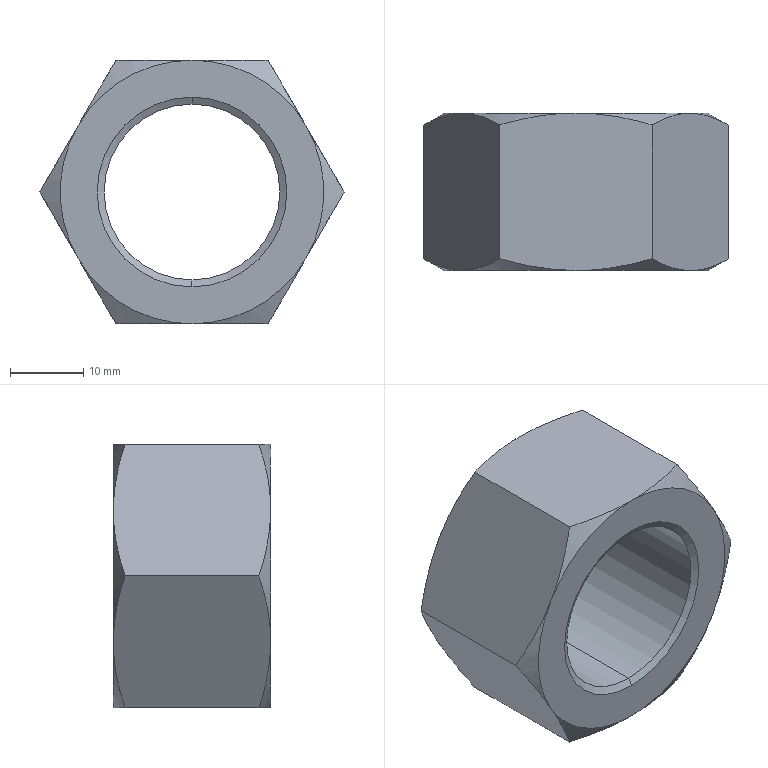Component | SolidWorks | GB_T6170-2015[Type1HexNutM24]-3 | 1 solid | 26 faces | box 41.57 x 21.5 x 36 mm | volume 14263 mm3 | cone 16 | plane 8 | cylinder 2 | commonest cylinder face diameters 24 x2
build123d program:
from build123d import *

# Parameters (mm, degrees)
SKETCH3_R               = 10.376
BOSS_EXTRUDE1_DEPTH     = 21.5
SKETCH5_R               = 29.663
SKETCH5_R_2             = 18
CUT_EXTRUDE1_2_DEPTH    = 4.3
CUT_EXTRUDE1_2_DRAFT    = -60
SKETCH7_R               = 29.663
SKETCH7_R_2             = 18
CUT_EXTRUDE2_DEPTH      = 4.3
CUT_EXTRUDE2_DRAFT      = -60
CUT_EXTRUDE1_DEPTH      = 35.903
CUT_EXTRUDE1_DEPTH_BACK = 35.903
SKETCH1_R               = 12


with BuildPart() as part:
    # Sketch3 → Boss-Extrude1 (new body)
    with BuildSketch(Plane.XY):
        Polygon((0, 20.785), (-18, 10.392), (-18, -10.392), (0, -20.785), (18, -10.392), (18, 10.392), align=None)
        Circle(SKETCH3_R, mode=Mode.SUBTRACT)
    extrude(amount=-BOSS_EXTRUDE1_DEPTH)

    # Sketch4 → Cut-Revolve1 (revolve, cut)
    with BuildSketch(Plane(origin=(0, 0, 0), x_dir=(0, 0, -1), z_dir=(1, 0, 0)), mode=Mode.PRIVATE) as cut_revolve1_sk:
        Polygon((0, 12.95), (1.486, 10.376), (1.486, 0), (0, 0), align=None)
        Polygon((21.5, 0), (21.5, 12.95), (20.014, 10.376), (20.014, 0), align=None)
    revolve(cut_revolve1_sk.sketch.rotate(Axis((0, 0, 0), (0, 0, -1)), 90), axis=Axis((0, 0, 0), (0, 0, -1)), mode=Mode.SUBTRACT)


with BuildPart() as cut_extrude1_2_tool:
    # Sketch5 → Cut-Extrude1_2 (with draft: the straight prism first)
    with BuildSketch(Plane.XY):
        Circle(SKETCH5_R)
        Circle(SKETCH5_R_2, mode=Mode.SUBTRACT)
    extrude(amount=-CUT_EXTRUDE1_2_DEPTH)
    # Cut-Extrude1_2: the draft: its side faces are tilted about the plane it starts from
    cut_extrude1_2_sides = [cut_extrude1_2_tool.faces().sort_by_distance(p)[0] for p in [
        (-29.663, 0, -2.15),
        (-18, 0, -2.15),
    ]]
    draft(cut_extrude1_2_sides, Plane.XY, CUT_EXTRUDE1_2_DRAFT)


with BuildPart() as part_1:
    add(part.part)

    # Cut-Extrude1_2: cut by cut_extrude1_2_tool
    add(cut_extrude1_2_tool.part, mode=Mode.SUBTRACT)


with BuildPart() as cut_extrude2_tool:
    # Sketch7 → Cut-Extrude2 (with draft: the straight prism first)
    with BuildSketch(Plane(origin=(0, 0, -21.5), x_dir=(-1, 0, 0), z_dir=(0, 0, -1))):
        Circle(SKETCH7_R)
        Circle(SKETCH7_R_2, mode=Mode.SUBTRACT)
    extrude(amount=-CUT_EXTRUDE2_DEPTH)
    # Cut-Extrude2: the draft: its side faces are tilted about the plane it starts from
    cut_extrude2_sides = [cut_extrude2_tool.faces().sort_by_distance(p)[0] for p in [
        (29.663, 0, -19.35),
        (18, 0, -19.35),
    ]]
    draft(cut_extrude2_sides, Plane(origin=(0, 0, -21.5), x_dir=(-1, 0, 0), z_dir=(0, 0, -1)), CUT_EXTRUDE2_DRAFT)


with BuildPart() as part_2:
    add(part_1.part)

    # Cut-Extrude2: cut by cut_extrude2_tool
    add(cut_extrude2_tool.part, mode=Mode.SUBTRACT)

    # Sketch1 → Cut-Extrude1 (cut, two sides: drawn at the far end of the back side and taken through both)
    with BuildSketch(Plane.XY.offset(-CUT_EXTRUDE1_DEPTH_BACK)):
        Circle(SKETCH1_R)
    extrude(amount=CUT_EXTRUDE1_DEPTH + CUT_EXTRUDE1_DEPTH_BACK, mode=Mode.SUBTRACT)


solid = part_2.part

# Placed as in the assembly
solid = solid.moved(Location((82.5, 20, 142.894), (90, 0, 90)))
STEP:
#1=COLOUR_RGB('',0.7922,0.8196,0.9333);
#2=FILL_AREA_STYLE_COLOUR('',#1);
#3=FILL_AREA_STYLE('',(#2));
#4=SURFACE_STYLE_FILL_AREA(#3);
#5=SURFACE_SIDE_STYLE('',(#4));
#6=SURFACE_STYLE_USAGE(.BOTH.,#5);
#7=PRESENTATION_STYLE_ASSIGNMENT((#6));
#8=CARTESIAN_POINT('',(3.248,0.809,5.153));
#9=VERTEX_POINT('',#8);
#10=CARTESIAN_POINT('',(3.248,0.809,6.098));
#11=VERTEX_POINT('',#10);
#12=CARTESIAN_POINT('',(3.248,0.809,5.626));
#13=DIRECTION('',(0.,-1.,0.));
#14=DIRECTION('',(0.,0.,1.));
#15=AXIS2_PLACEMENT_3D('',#12,#13,#14);
#16=CIRCLE('',#15,0.4724);
#17=EDGE_CURVE('',#9,#11,#16,.T.);
#18=ORIENTED_EDGE('',*,*,#17,.T.);
#19=CARTESIAN_POINT('',(3.248,1.612,6.098));
#20=VERTEX_POINT('',#19);
#21=CARTESIAN_POINT('',(3.248,0.7874,6.098));
#22=DIRECTION('',(0.,1.,0.));
#23=VECTOR('',#22,39.37);
#24=LINE('',#21,#23);
#25=EDGE_CURVE('',#11,#20,#24,.T.);
#26=ORIENTED_EDGE('',*,*,#25,.T.);
#27=CARTESIAN_POINT('',(3.248,1.612,5.153));
#28=VERTEX_POINT('',#27);
#29=CARTESIAN_POINT('',(3.248,1.612,5.626));
#30=DIRECTION('',(0.,1.,0.));
#31=DIRECTION('',(-0.,0.,-1.));
#32=AXIS2_PLACEMENT_3D('',#29,#30,#31);
#33=CIRCLE('',#32,0.4724);
#34=EDGE_CURVE('',#20,#28,#33,.T.);
#35=ORIENTED_EDGE('',*,*,#34,.T.);
#36=CARTESIAN_POINT('',(3.248,0.7874,5.153));
#37=DIRECTION('',(0.,1.,0.));
#38=VECTOR('',#37,39.37);
#39=LINE('',#36,#38);
#40=EDGE_CURVE('',#9,#28,#39,.T.);
#41=ORIENTED_EDGE('',*,*,#40,.F.);
#42=EDGE_LOOP('',(#18,#26,#35,#41));
#43=FACE_OUTER_BOUND('',#42,.T.);
#44=CARTESIAN_POINT('',(3.248,0.7874,5.626));
#45=DIRECTION('',(0.,1.,0.));
#46=DIRECTION('',(-0.,0.,-1.));
#47=AXIS2_PLACEMENT_3D('',#44,#45,#46);
#48=CYLINDRICAL_SURFACE('',#47,0.4724);
#49=ADVANCED_FACE('',(#43),#48,.F.);
#50=ORIENTED_EDGE('',*,*,#17,.F.);
#51=CARTESIAN_POINT('',(3.248,0.7874,5.116));
#52=VERTEX_POINT('',#51);
#53=CARTESIAN_POINT('',(3.248,0.7874,5.116));
#54=DIRECTION('',(-0.,-0.5,-0.866));
#55=VECTOR('',#54,39.37);
#56=LINE('',#53,#55);
#57=EDGE_CURVE('',#9,#52,#56,.T.);
#58=ORIENTED_EDGE('',*,*,#57,.T.);
#59=CARTESIAN_POINT('',(3.248,0.7874,6.136));
#60=VERTEX_POINT('',#59);
#61=CARTESIAN_POINT('',(3.248,0.7874,5.626));
#62=DIRECTION('',(0.,1.,0.));
#63=DIRECTION('',(-0.,0.,-1.));
#64=AXIS2_PLACEMENT_3D('',#61,#62,#63);
#65=CIRCLE('',#64,0.5098);
#66=EDGE_CURVE('',#60,#52,#65,.T.);
#67=ORIENTED_EDGE('',*,*,#66,.F.);
#68=CARTESIAN_POINT('',(3.248,0.7874,6.136));
#69=DIRECTION('',(0.,-0.5,0.866));
#70=VECTOR('',#69,39.37);
#71=LINE('',#68,#70);
#72=EDGE_CURVE('',#11,#60,#71,.T.);
#73=ORIENTED_EDGE('',*,*,#72,.F.);
#74=EDGE_LOOP('',(#50,#58,#67,#73));
#75=FACE_OUTER_BOUND('',#74,.T.);
#76=CARTESIAN_POINT('',(3.248,0.7874,5.626));
#77=DIRECTION('',(0.,-1.,0.));
#78=DIRECTION('',(0.,0.,1.));
#79=AXIS2_PLACEMENT_3D('',#76,#77,#78);
#80=CONICAL_SURFACE('',#79,0.5098,1.047);
#81=ADVANCED_FACE('',(#75),#80,.F.);
#82=ORIENTED_EDGE('',*,*,#34,.F.);
#83=CARTESIAN_POINT('',(3.248,1.634,6.136));
#84=VERTEX_POINT('',#83);
#85=CARTESIAN_POINT('',(3.248,1.575,6.034));
#86=DIRECTION('',(0.,0.5,0.866));
#87=VECTOR('',#86,39.37);
#88=LINE('',#85,#87);
#89=EDGE_CURVE('',#20,#84,#88,.T.);
#90=ORIENTED_EDGE('',*,*,#89,.T.);
#91=CARTESIAN_POINT('',(3.248,1.634,5.116));
#92=VERTEX_POINT('',#91);
#93=CARTESIAN_POINT('',(3.248,1.634,5.626));
#94=DIRECTION('',(0.,1.,0.));
#95=DIRECTION('',(-0.,0.,-1.));
#96=AXIS2_PLACEMENT_3D('',#93,#94,#95);
#97=CIRCLE('',#96,0.5098);
#98=EDGE_CURVE('',#84,#92,#97,.T.);
#99=ORIENTED_EDGE('',*,*,#98,.T.);
#100=CARTESIAN_POINT('',(3.248,1.575,5.217));
#101=DIRECTION('',(-0.,0.5,-0.866));
#102=VECTOR('',#101,39.37);
#103=LINE('',#100,#102);
#104=EDGE_CURVE('',#28,#92,#103,.T.);
#105=ORIENTED_EDGE('',*,*,#104,.F.);
#106=EDGE_LOOP('',(#82,#90,#99,#105));
#107=FACE_OUTER_BOUND('',#106,.T.);
#108=CARTESIAN_POINT('',(3.248,1.575,5.626));
#109=DIRECTION('',(0.,1.,0.));
#110=DIRECTION('',(-0.,0.,-1.));
#111=AXIS2_PLACEMENT_3D('',#108,#109,#110);
#112=CONICAL_SURFACE('',#111,0.4085,1.047);
#113=ADVANCED_FACE('',(#107),#112,.F.);
#114=CARTESIAN_POINT('',(2.839,0.8507,4.917));
#115=VERTEX_POINT('',#114);
#116=CARTESIAN_POINT('',(2.839,1.571,4.917));
#117=VERTEX_POINT('',#116);
#118=CARTESIAN_POINT('',(2.839,0.7874,4.917));
#119=DIRECTION('',(0.,1.,0.));
#120=VECTOR('',#119,39.37);
#121=LINE('',#118,#120);
#122=EDGE_CURVE('',#115,#117,#121,.T.);
#123=ORIENTED_EDGE('',*,*,#122,.F.);
#124=CARTESIAN_POINT('',(2.634,0.7874,5.271));
#125=VERTEX_POINT('',#124);
#126=CARTESIAN_POINT('',(2.839,0.8507,4.917));
#127=CARTESIAN_POINT('',(2.805,0.8314,4.975));
#128=CARTESIAN_POINT('',(2.772,0.8155,5.033));
#129=CARTESIAN_POINT('',(2.704,0.7934,5.151));
#130=CARTESIAN_POINT('',(2.669,0.7874,5.211));
#131=CARTESIAN_POINT('',(2.634,0.7874,5.271));
#132=B_SPLINE_CURVE_WITH_KNOTS('',3,(#126,#127,#128,#129,#130,#131),.UNSPECIFIED.,.F.,.F.,(4,2,4),(0.00000024,0.005258,0.01052),.UNSPECIFIED.);
#133=EDGE_CURVE('',#115,#125,#132,.T.);
#134=ORIENTED_EDGE('',*,*,#133,.T.);
#135=CARTESIAN_POINT('',(2.43,0.8507,5.626));
#136=VERTEX_POINT('',#135);
#137=CARTESIAN_POINT('',(2.634,0.7874,5.271));
#138=CARTESIAN_POINT('',(2.626,0.7874,5.286));
#139=CARTESIAN_POINT('',(2.617,0.7878,5.302));
#140=CARTESIAN_POINT('',(2.6,0.7892,5.332));
#141=CARTESIAN_POINT('',(2.591,0.7903,5.347));
#142=CARTESIAN_POINT('',(2.565,0.7947,5.391));
#143=CARTESIAN_POINT('',(2.548,0.799,5.421));
#144=CARTESIAN_POINT('',(2.497,0.8155,5.51));
#145=CARTESIAN_POINT('',(2.463,0.8314,5.568));
#146=CARTESIAN_POINT('',(2.43,0.8507,5.626));
#147=B_SPLINE_CURVE_WITH_KNOTS('',3,(#137,#138,#139,#140,#141,#142,#143,#144,#145,#146),.UNSPECIFIED.,.F.,.F.,(4,2,2,2,4),(0.01052,0.01183,0.01313,0.01575,0.02099),.UNSPECIFIED.);
#148=EDGE_CURVE('',#125,#136,#147,.T.);
#149=ORIENTED_EDGE('',*,*,#148,.T.);
#150=CARTESIAN_POINT('',(2.43,1.571,5.626));
#151=VERTEX_POINT('',#150);
#152=CARTESIAN_POINT('',(2.43,0.7874,5.626));
#153=DIRECTION('',(0.,1.,0.));
#154=VECTOR('',#153,39.37);
#155=LINE('',#152,#154);
#156=EDGE_CURVE('',#136,#151,#155,.T.);
#157=ORIENTED_EDGE('',*,*,#156,.T.);
#158=CARTESIAN_POINT('',(2.634,1.634,5.271));
#159=VERTEX_POINT('',#158);
#160=CARTESIAN_POINT('',(2.43,1.571,5.626));
#161=CARTESIAN_POINT('',(2.463,1.59,5.568));
#162=CARTESIAN_POINT('',(2.497,1.606,5.509));
#163=CARTESIAN_POINT('',(2.565,1.628,5.391));
#164=CARTESIAN_POINT('',(2.599,1.634,5.332));
#165=CARTESIAN_POINT('',(2.634,1.634,5.271));
#166=B_SPLINE_CURVE_WITH_KNOTS('',3,(#160,#161,#162,#163,#164,#165),.UNSPECIFIED.,.F.,.F.,(4,2,4),(0.00000024,0.005258,0.01052),.UNSPECIFIED.);
#167=EDGE_CURVE('',#151,#159,#166,.T.);
#168=ORIENTED_EDGE('',*,*,#167,.T.);
#169=CARTESIAN_POINT('',(2.634,1.634,5.271));
#170=CARTESIAN_POINT('',(2.643,1.634,5.256));
#171=CARTESIAN_POINT('',(2.652,1.633,5.241));
#172=CARTESIAN_POINT('',(2.669,1.632,5.211));
#173=CARTESIAN_POINT('',(2.678,1.631,5.196));
#174=CARTESIAN_POINT('',(2.704,1.627,5.151));
#175=CARTESIAN_POINT('',(2.721,1.622,5.122));
#176=CARTESIAN_POINT('',(2.772,1.606,5.033));
#177=CARTESIAN_POINT('',(2.806,1.59,4.975));
#178=CARTESIAN_POINT('',(2.839,1.571,4.917));
#179=B_SPLINE_CURVE_WITH_KNOTS('',3,(#169,#170,#171,#172,#173,#174,#175,#176,#177,#178),.UNSPECIFIED.,.F.,.F.,(4,2,2,2,4),(0.01052,0.01183,0.01313,0.01575,0.02099),.UNSPECIFIED.);
#180=EDGE_CURVE('',#159,#117,#179,.T.);
#181=ORIENTED_EDGE('',*,*,#180,.T.);
#182=EDGE_LOOP('',(#123,#134,#149,#157,#168,#181));
#183=FACE_OUTER_BOUND('',#182,.T.);
#184=CARTESIAN_POINT('',(2.839,0.7874,4.917));
#185=DIRECTION('',(-0.866,0.,-0.5));
#186=DIRECTION('',(-0.5,0.,0.866));
#187=AXIS2_PLACEMENT_3D('',#184,#185,#186);
#188=PLANE('',#187);
#189=ADVANCED_FACE('',(#183),#188,.T.);
#190=CARTESIAN_POINT('',(3.657,0.8507,4.917));
#191=VERTEX_POINT('',#190);
#192=CARTESIAN_POINT('',(3.657,1.571,4.917));
#193=VERTEX_POINT('',#192);
#194=CARTESIAN_POINT('',(3.657,0.7874,4.917));
#195=DIRECTION('',(0.,1.,0.));
#196=VECTOR('',#195,39.37);
#197=LINE('',#194,#196);
#198=EDGE_CURVE('',#191,#193,#197,.T.);
#199=ORIENTED_EDGE('',*,*,#198,.F.);
#200=CARTESIAN_POINT('',(3.248,0.7874,4.917));
#201=VERTEX_POINT('',#200);
#202=CARTESIAN_POINT('',(3.657,0.8507,4.917));
#203=CARTESIAN_POINT('',(3.591,0.8315,4.917));
#204=CARTESIAN_POINT('',(3.522,0.8154,4.917));
#205=CARTESIAN_POINT('',(3.386,0.7933,4.917));
#206=CARTESIAN_POINT('',(3.317,0.7874,4.917));
#207=CARTESIAN_POINT('',(3.248,0.7874,4.917));
#208=B_SPLINE_CURVE_WITH_KNOTS('',3,(#202,#203,#204,#205,#206,#207),.UNSPECIFIED.,.F.,.F.,(4,2,4),(0.01881,0.02407,0.02933),.UNSPECIFIED.);
#209=EDGE_CURVE('',#191,#201,#208,.T.);
#210=ORIENTED_EDGE('',*,*,#209,.T.);
#211=CARTESIAN_POINT('',(3.248,0.7874,4.917));
#212=CARTESIAN_POINT('',(3.213,0.7874,4.917));
#213=CARTESIAN_POINT('',(3.179,0.7889,4.917));
#214=CARTESIAN_POINT('',(3.109,0.7947,4.917));
#215=CARTESIAN_POINT('',(3.075,0.7991,4.917));
#216=CARTESIAN_POINT('',(2.972,0.8157,4.917));
#217=CARTESIAN_POINT('',(2.905,0.8316,4.917));
#218=CARTESIAN_POINT('',(2.839,0.8507,4.917));
#219=B_SPLINE_CURVE_WITH_KNOTS('',3,(#211,#212,#213,#214,#215,#216,#217,#218),.UNSPECIFIED.,.F.,.F.,(4,2,2,4),(0.02933,0.03196,0.03459,0.03985),.UNSPECIFIED.);
#220=EDGE_CURVE('',#201,#115,#219,.T.);
#221=ORIENTED_EDGE('',*,*,#220,.T.);
#222=ORIENTED_EDGE('',*,*,#122,.T.);
#223=CARTESIAN_POINT('',(3.248,1.634,4.917));
#224=VERTEX_POINT('',#223);
#225=CARTESIAN_POINT('',(2.839,1.571,4.917));
#226=CARTESIAN_POINT('',(2.905,1.59,4.917));
#227=CARTESIAN_POINT('',(2.972,1.606,4.917));
#228=CARTESIAN_POINT('',(3.075,1.622,4.917));
#229=CARTESIAN_POINT('',(3.109,1.627,4.917));
#230=CARTESIAN_POINT('',(3.179,1.632,4.917));
#231=CARTESIAN_POINT('',(3.213,1.634,4.917));
#232=CARTESIAN_POINT('',(3.248,1.634,4.917));
#233=B_SPLINE_CURVE_WITH_KNOTS('',3,(#225,#226,#227,#228,#229,#230,#231,#232),.UNSPECIFIED.,.F.,.F.,(4,2,2,4),(0.04624,0.05151,0.05414,0.05678),.UNSPECIFIED.);
#234=EDGE_CURVE('',#117,#224,#233,.T.);
#235=ORIENTED_EDGE('',*,*,#234,.T.);
#236=CARTESIAN_POINT('',(3.248,1.634,4.917));
#237=CARTESIAN_POINT('',(3.317,1.634,4.917));
#238=CARTESIAN_POINT('',(3.386,1.628,4.917));
#239=CARTESIAN_POINT('',(3.522,1.606,4.917));
#240=CARTESIAN_POINT('',(3.591,1.59,4.917));
#241=CARTESIAN_POINT('',(3.657,1.571,4.917));
#242=B_SPLINE_CURVE_WITH_KNOTS('',3,(#236,#237,#238,#239,#240,#241),.UNSPECIFIED.,.F.,.F.,(4,2,4),(0.05678,0.06204,0.0673),.UNSPECIFIED.);
#243=EDGE_CURVE('',#224,#193,#242,.T.);
#244=ORIENTED_EDGE('',*,*,#243,.T.);
#245=EDGE_LOOP('',(#199,#210,#221,#222,#235,#244));
#246=FACE_OUTER_BOUND('',#245,.T.);
#247=CARTESIAN_POINT('',(3.657,0.7874,4.917));
#248=DIRECTION('',(-0.,0.,-1.));
#249=DIRECTION('',(-1.,0.,0.));
#250=AXIS2_PLACEMENT_3D('',#247,#248,#249);
#251=PLANE('',#250);
#252=ADVANCED_FACE('',(#246),#251,.T.);
#253=CARTESIAN_POINT('',(4.066,0.8507,5.626));
#254=VERTEX_POINT('',#253);
#255=CARTESIAN_POINT('',(4.066,1.571,5.626));
#256=VERTEX_POINT('',#255);
#257=CARTESIAN_POINT('',(4.066,0.7874,5.626));
#258=DIRECTION('',(0.,1.,0.));
#259=VECTOR('',#258,39.37);
#260=LINE('',#257,#259);
#261=EDGE_CURVE('',#254,#256,#260,.T.);
#262=ORIENTED_EDGE('',*,*,#261,.F.);
#263=CARTESIAN_POINT('',(3.862,0.7874,5.271));
#264=VERTEX_POINT('',#263);
#265=CARTESIAN_POINT('',(4.066,0.8507,5.626));
#266=CARTESIAN_POINT('',(4.033,0.8314,5.568));
#267=CARTESIAN_POINT('',(3.999,0.8155,5.509));
#268=CARTESIAN_POINT('',(3.931,0.7934,5.391));
#269=CARTESIAN_POINT('',(3.897,0.7874,5.332));
#270=CARTESIAN_POINT('',(3.862,0.7874,5.271));
#271=B_SPLINE_CURVE_WITH_KNOTS('',3,(#265,#266,#267,#268,#269,#270),.UNSPECIFIED.,.F.,.F.,(4,2,4),(0.00000024,0.005258,0.01052),.UNSPECIFIED.);
#272=EDGE_CURVE('',#254,#264,#271,.T.);
#273=ORIENTED_EDGE('',*,*,#272,.T.);
#274=CARTESIAN_POINT('',(3.862,0.7874,5.271));
#275=CARTESIAN_POINT('',(3.853,0.7874,5.256));
#276=CARTESIAN_POINT('',(3.844,0.7878,5.241));
#277=CARTESIAN_POINT('',(3.827,0.7892,5.211));
#278=CARTESIAN_POINT('',(3.818,0.7903,5.196));
#279=CARTESIAN_POINT('',(3.792,0.7947,5.151));
#280=CARTESIAN_POINT('',(3.775,0.799,5.122));
#281=CARTESIAN_POINT('',(3.724,0.8155,5.033));
#282=CARTESIAN_POINT('',(3.691,0.8314,4.975));
#283=CARTESIAN_POINT('',(3.657,0.8507,4.917));
#284=B_SPLINE_CURVE_WITH_KNOTS('',3,(#274,#275,#276,#277,#278,#279,#280,#281,#282,#283),.UNSPECIFIED.,.F.,.F.,(4,2,2,2,4),(0.01052,0.01183,0.01313,0.01575,0.02099),.UNSPECIFIED.);
#285=EDGE_CURVE('',#264,#191,#284,.T.);
#286=ORIENTED_EDGE('',*,*,#285,.T.);
#287=ORIENTED_EDGE('',*,*,#198,.T.);
#288=CARTESIAN_POINT('',(3.862,1.634,5.271));
#289=VERTEX_POINT('',#288);
#290=CARTESIAN_POINT('',(3.657,1.571,4.917));
#291=CARTESIAN_POINT('',(3.691,1.59,4.975));
#292=CARTESIAN_POINT('',(3.724,1.606,5.033));
#293=CARTESIAN_POINT('',(3.792,1.628,5.151));
#294=CARTESIAN_POINT('',(3.827,1.634,5.211));
#295=CARTESIAN_POINT('',(3.862,1.634,5.271));
#296=B_SPLINE_CURVE_WITH_KNOTS('',3,(#290,#291,#292,#293,#294,#295),.UNSPECIFIED.,.F.,.F.,(4,2,4),(0.00000024,0.005258,0.01052),.UNSPECIFIED.);
#297=EDGE_CURVE('',#193,#289,#296,.T.);
#298=ORIENTED_EDGE('',*,*,#297,.T.);
#299=CARTESIAN_POINT('',(3.862,1.634,5.271));
#300=CARTESIAN_POINT('',(3.87,1.634,5.286));
#301=CARTESIAN_POINT('',(3.879,1.633,5.302));
#302=CARTESIAN_POINT('',(3.897,1.632,5.332));
#303=CARTESIAN_POINT('',(3.905,1.631,5.347));
#304=CARTESIAN_POINT('',(3.931,1.627,5.391));
#305=CARTESIAN_POINT('',(3.948,1.622,5.421));
#306=CARTESIAN_POINT('',(3.999,1.606,5.51));
#307=CARTESIAN_POINT('',(4.033,1.59,5.568));
#308=CARTESIAN_POINT('',(4.066,1.571,5.626));
#309=B_SPLINE_CURVE_WITH_KNOTS('',3,(#299,#300,#301,#302,#303,#304,#305,#306,#307,#308),.UNSPECIFIED.,.F.,.F.,(4,2,2,2,4),(0.01052,0.01183,0.01313,0.01575,0.02099),.UNSPECIFIED.);
#310=EDGE_CURVE('',#289,#256,#309,.T.);
#311=ORIENTED_EDGE('',*,*,#310,.T.);
#312=EDGE_LOOP('',(#262,#273,#286,#287,#298,#311));
#313=FACE_OUTER_BOUND('',#312,.T.);
#314=CARTESIAN_POINT('',(4.066,0.7874,5.626));
#315=DIRECTION('',(0.866,0.,-0.5));
#316=DIRECTION('',(-0.5,0.,-0.866));
#317=AXIS2_PLACEMENT_3D('',#314,#315,#316);
#318=PLANE('',#317);
#319=ADVANCED_FACE('',(#313),#318,.T.);
#320=CARTESIAN_POINT('',(3.657,0.8507,6.334));
#321=VERTEX_POINT('',#320);
#322=CARTESIAN_POINT('',(3.657,1.571,6.334));
#323=VERTEX_POINT('',#322);
#324=CARTESIAN_POINT('',(3.657,0.7874,6.334));
#325=DIRECTION('',(0.,1.,0.));
#326=VECTOR('',#325,39.37);
#327=LINE('',#324,#326);
#328=EDGE_CURVE('',#321,#323,#327,.T.);
#329=ORIENTED_EDGE('',*,*,#328,.F.);
#330=CARTESIAN_POINT('',(3.862,0.7874,5.98));
#331=VERTEX_POINT('',#330);
#332=CARTESIAN_POINT('',(3.657,0.8507,6.334));
#333=CARTESIAN_POINT('',(3.691,0.8314,6.276));
#334=CARTESIAN_POINT('',(3.724,0.8155,6.218));
#335=CARTESIAN_POINT('',(3.792,0.7934,6.1));
#336=CARTESIAN_POINT('',(3.827,0.7874,6.04));
#337=CARTESIAN_POINT('',(3.862,0.7874,5.98));
#338=B_SPLINE_CURVE_WITH_KNOTS('',3,(#332,#333,#334,#335,#336,#337),.UNSPECIFIED.,.F.,.F.,(4,2,4),(0.00000024,0.005258,0.01052),.UNSPECIFIED.);
#339=EDGE_CURVE('',#321,#331,#338,.T.);
#340=ORIENTED_EDGE('',*,*,#339,.T.);
#341=CARTESIAN_POINT('',(3.862,0.7874,5.98));
#342=CARTESIAN_POINT('',(3.87,0.7874,5.965));
#343=CARTESIAN_POINT('',(3.879,0.7878,5.95));
#344=CARTESIAN_POINT('',(3.897,0.7892,5.92));
#345=CARTESIAN_POINT('',(3.905,0.7903,5.905));
#346=CARTESIAN_POINT('',(3.931,0.7947,5.86));
#347=CARTESIAN_POINT('',(3.948,0.799,5.83));
#348=CARTESIAN_POINT('',(3.999,0.8155,5.742));
#349=CARTESIAN_POINT('',(4.033,0.8314,5.684));
#350=CARTESIAN_POINT('',(4.066,0.8507,5.626));
#351=B_SPLINE_CURVE_WITH_KNOTS('',3,(#341,#342,#343,#344,#345,#346,#347,#348,#349,#350),.UNSPECIFIED.,.F.,.F.,(4,2,2,2,4),(0.01052,0.01183,0.01313,0.01575,0.02099),.UNSPECIFIED.);
#352=EDGE_CURVE('',#331,#254,#351,.T.);
#353=ORIENTED_EDGE('',*,*,#352,.T.);
#354=ORIENTED_EDGE('',*,*,#261,.T.);
#355=CARTESIAN_POINT('',(3.862,1.634,5.98));
#356=VERTEX_POINT('',#355);
#357=CARTESIAN_POINT('',(4.066,1.571,5.626));
#358=CARTESIAN_POINT('',(4.033,1.59,5.684));
#359=CARTESIAN_POINT('',(3.999,1.606,5.742));
#360=CARTESIAN_POINT('',(3.931,1.628,5.86));
#361=CARTESIAN_POINT('',(3.897,1.634,5.92));
#362=CARTESIAN_POINT('',(3.862,1.634,5.98));
#363=B_SPLINE_CURVE_WITH_KNOTS('',3,(#357,#358,#359,#360,#361,#362),.UNSPECIFIED.,.F.,.F.,(4,2,4),(0.00000024,0.005258,0.01052),.UNSPECIFIED.);
#364=EDGE_CURVE('',#256,#356,#363,.T.);
#365=ORIENTED_EDGE('',*,*,#364,.T.);
#366=CARTESIAN_POINT('',(3.862,1.634,5.98));
#367=CARTESIAN_POINT('',(3.853,1.634,5.995));
#368=CARTESIAN_POINT('',(3.844,1.633,6.01));
#369=CARTESIAN_POINT('',(3.827,1.632,6.04));
#370=CARTESIAN_POINT('',(3.818,1.631,6.055));
#371=CARTESIAN_POINT('',(3.792,1.627,6.1));
#372=CARTESIAN_POINT('',(3.775,1.622,6.13));
#373=CARTESIAN_POINT('',(3.724,1.606,6.218));
#374=CARTESIAN_POINT('',(3.691,1.59,6.277));
#375=CARTESIAN_POINT('',(3.657,1.571,6.334));
#376=B_SPLINE_CURVE_WITH_KNOTS('',3,(#366,#367,#368,#369,#370,#371,#372,#373,#374,#375),.UNSPECIFIED.,.F.,.F.,(4,2,2,2,4),(0.01052,0.01183,0.01313,0.01575,0.02099),.UNSPECIFIED.);
#377=EDGE_CURVE('',#356,#323,#376,.T.);
#378=ORIENTED_EDGE('',*,*,#377,.T.);
#379=EDGE_LOOP('',(#329,#340,#353,#354,#365,#378));
#380=FACE_OUTER_BOUND('',#379,.T.);
#381=CARTESIAN_POINT('',(3.657,0.7874,6.334));
#382=DIRECTION('',(0.866,0.,0.5));
#383=DIRECTION('',(0.5,0.,-0.866));
#384=AXIS2_PLACEMENT_3D('',#381,#382,#383);
#385=PLANE('',#384);
#386=ADVANCED_FACE('',(#380),#385,.T.);
#387=CARTESIAN_POINT('',(2.839,0.8507,6.334));
#388=VERTEX_POINT('',#387);
#389=CARTESIAN_POINT('',(2.839,1.571,6.334));
#390=VERTEX_POINT('',#389);
#391=CARTESIAN_POINT('',(2.839,0.7874,6.334));
#392=DIRECTION('',(0.,1.,0.));
#393=VECTOR('',#392,39.37);
#394=LINE('',#391,#393);
#395=EDGE_CURVE('',#388,#390,#394,.T.);
#396=ORIENTED_EDGE('',*,*,#395,.F.);
#397=CARTESIAN_POINT('',(3.248,0.7874,6.334));
#398=VERTEX_POINT('',#397);
#399=CARTESIAN_POINT('',(2.839,0.8507,6.334));
#400=CARTESIAN_POINT('',(2.905,0.8316,6.334));
#401=CARTESIAN_POINT('',(2.972,0.8157,6.334));
#402=CARTESIAN_POINT('',(3.075,0.7991,6.334));
#403=CARTESIAN_POINT('',(3.109,0.7947,6.334));
#404=CARTESIAN_POINT('',(3.179,0.7889,6.334));
#405=CARTESIAN_POINT('',(3.213,0.7874,6.334));
#406=CARTESIAN_POINT('',(3.248,0.7874,6.334));
#407=B_SPLINE_CURVE_WITH_KNOTS('',3,(#399,#400,#401,#402,#403,#404,#405,#406),.UNSPECIFIED.,.F.,.F.,(4,2,2,4),(0.04624,0.05151,0.05414,0.05678),.UNSPECIFIED.);
#408=EDGE_CURVE('',#388,#398,#407,.T.);
#409=ORIENTED_EDGE('',*,*,#408,.T.);
#410=CARTESIAN_POINT('',(3.248,0.7874,6.334));
#411=CARTESIAN_POINT('',(3.317,0.7874,6.334));
#412=CARTESIAN_POINT('',(3.386,0.7933,6.334));
#413=CARTESIAN_POINT('',(3.522,0.8154,6.334));
#414=CARTESIAN_POINT('',(3.591,0.8315,6.334));
#415=CARTESIAN_POINT('',(3.657,0.8507,6.334));
#416=B_SPLINE_CURVE_WITH_KNOTS('',3,(#410,#411,#412,#413,#414,#415),.UNSPECIFIED.,.F.,.F.,(4,2,4),(0.05678,0.06204,0.0673),.UNSPECIFIED.);
#417=EDGE_CURVE('',#398,#321,#416,.T.);
#418=ORIENTED_EDGE('',*,*,#417,.T.);
#419=ORIENTED_EDGE('',*,*,#328,.T.);
#420=CARTESIAN_POINT('',(3.248,1.634,6.334));
#421=VERTEX_POINT('',#420);
#422=CARTESIAN_POINT('',(3.657,1.571,6.334));
#423=CARTESIAN_POINT('',(3.591,1.59,6.334));
#424=CARTESIAN_POINT('',(3.522,1.606,6.334));
#425=CARTESIAN_POINT('',(3.386,1.628,6.334));
#426=CARTESIAN_POINT('',(3.317,1.634,6.334));
#427=CARTESIAN_POINT('',(3.248,1.634,6.334));
#428=B_SPLINE_CURVE_WITH_KNOTS('',3,(#422,#423,#424,#425,#426,#427),.UNSPECIFIED.,.F.,.F.,(4,2,4),(0.01881,0.02407,0.02933),.UNSPECIFIED.);
#429=EDGE_CURVE('',#323,#421,#428,.T.);
#430=ORIENTED_EDGE('',*,*,#429,.T.);
#431=CARTESIAN_POINT('',(3.248,1.634,6.334));
#432=CARTESIAN_POINT('',(3.213,1.634,6.334));
#433=CARTESIAN_POINT('',(3.179,1.632,6.334));
#434=CARTESIAN_POINT('',(3.109,1.627,6.334));
#435=CARTESIAN_POINT('',(3.075,1.622,6.334));
#436=CARTESIAN_POINT('',(2.972,1.606,6.334));
#437=CARTESIAN_POINT('',(2.905,1.59,6.334));
#438=CARTESIAN_POINT('',(2.839,1.571,6.334));
#439=B_SPLINE_CURVE_WITH_KNOTS('',3,(#431,#432,#433,#434,#435,#436,#437,#438),.UNSPECIFIED.,.F.,.F.,(4,2,2,4),(0.02933,0.03196,0.03459,0.03985),.UNSPECIFIED.);
#440=EDGE_CURVE('',#421,#390,#439,.T.);
#441=ORIENTED_EDGE('',*,*,#440,.T.);
#442=EDGE_LOOP('',(#396,#409,#418,#419,#430,#441));
#443=FACE_OUTER_BOUND('',#442,.T.);
#444=CARTESIAN_POINT('',(2.839,0.7874,6.334));
#445=DIRECTION('',(0.,0.,1.));
#446=DIRECTION('',(1.,0.,-0.));
#447=AXIS2_PLACEMENT_3D('',#444,#445,#446);
#448=PLANE('',#447);
#449=ADVANCED_FACE('',(#443),#448,.T.);
#450=ORIENTED_EDGE('',*,*,#156,.F.);
#451=CARTESIAN_POINT('',(2.634,0.7874,5.98));
#452=VERTEX_POINT('',#451);
#453=CARTESIAN_POINT('',(2.43,0.8507,5.626));
#454=CARTESIAN_POINT('',(2.463,0.8314,5.684));
#455=CARTESIAN_POINT('',(2.497,0.8155,5.742));
#456=CARTESIAN_POINT('',(2.565,0.7934,5.86));
#457=CARTESIAN_POINT('',(2.599,0.7874,5.92));
#458=CARTESIAN_POINT('',(2.634,0.7874,5.98));
#459=B_SPLINE_CURVE_WITH_KNOTS('',3,(#453,#454,#455,#456,#457,#458),.UNSPECIFIED.,.F.,.F.,(4,2,4),(0.00000024,0.005258,0.01052),.UNSPECIFIED.);
#460=EDGE_CURVE('',#136,#452,#459,.T.);
#461=ORIENTED_EDGE('',*,*,#460,.T.);
#462=CARTESIAN_POINT('',(2.634,0.7874,5.98));
#463=CARTESIAN_POINT('',(2.643,0.7874,5.995));
#464=CARTESIAN_POINT('',(2.652,0.7878,6.01));
#465=CARTESIAN_POINT('',(2.669,0.7892,6.04));
#466=CARTESIAN_POINT('',(2.678,0.7903,6.055));
#467=CARTESIAN_POINT('',(2.704,0.7947,6.1));
#468=CARTESIAN_POINT('',(2.721,0.799,6.13));
#469=CARTESIAN_POINT('',(2.772,0.8155,6.218));
#470=CARTESIAN_POINT('',(2.806,0.8314,6.277));
#471=CARTESIAN_POINT('',(2.839,0.8507,6.334));
#472=B_SPLINE_CURVE_WITH_KNOTS('',3,(#462,#463,#464,#465,#466,#467,#468,#469,#470,#471),.UNSPECIFIED.,.F.,.F.,(4,2,2,2,4),(0.01052,0.01183,0.01313,0.01575,0.02099),.UNSPECIFIED.);
#473=EDGE_CURVE('',#452,#388,#472,.T.);
#474=ORIENTED_EDGE('',*,*,#473,.T.);
#475=ORIENTED_EDGE('',*,*,#395,.T.);
#476=CARTESIAN_POINT('',(2.634,1.634,5.98));
#477=VERTEX_POINT('',#476);
#478=CARTESIAN_POINT('',(2.839,1.571,6.334));
#479=CARTESIAN_POINT('',(2.805,1.59,6.276));
#480=CARTESIAN_POINT('',(2.772,1.606,6.218));
#481=CARTESIAN_POINT('',(2.704,1.628,6.1));
#482=CARTESIAN_POINT('',(2.669,1.634,6.04));
#483=CARTESIAN_POINT('',(2.634,1.634,5.98));
#484=B_SPLINE_CURVE_WITH_KNOTS('',3,(#478,#479,#480,#481,#482,#483),.UNSPECIFIED.,.F.,.F.,(4,2,4),(0.00000024,0.005258,0.01052),.UNSPECIFIED.);
#485=EDGE_CURVE('',#390,#477,#484,.T.);
#486=ORIENTED_EDGE('',*,*,#485,.T.);
#487=CARTESIAN_POINT('',(2.634,1.634,5.98));
#488=CARTESIAN_POINT('',(2.626,1.634,5.965));
#489=CARTESIAN_POINT('',(2.617,1.633,5.95));
#490=CARTESIAN_POINT('',(2.6,1.632,5.92));
#491=CARTESIAN_POINT('',(2.591,1.631,5.905));
#492=CARTESIAN_POINT('',(2.565,1.627,5.86));
#493=CARTESIAN_POINT('',(2.548,1.622,5.83));
#494=CARTESIAN_POINT('',(2.497,1.606,5.742));
#495=CARTESIAN_POINT('',(2.463,1.59,5.684));
#496=CARTESIAN_POINT('',(2.43,1.571,5.626));
#497=B_SPLINE_CURVE_WITH_KNOTS('',3,(#487,#488,#489,#490,#491,#492,#493,#494,#495,#496),.UNSPECIFIED.,.F.,.F.,(4,2,2,2,4),(0.01052,0.01183,0.01313,0.01575,0.02099),.UNSPECIFIED.);
#498=EDGE_CURVE('',#477,#151,#497,.T.);
#499=ORIENTED_EDGE('',*,*,#498,.T.);
#500=EDGE_LOOP('',(#450,#461,#474,#475,#486,#499));
#501=FACE_OUTER_BOUND('',#500,.T.);
#502=CARTESIAN_POINT('',(2.43,0.7874,5.626));
#503=DIRECTION('',(-0.866,0.,0.5));
#504=DIRECTION('',(0.5,0.,0.866));
#505=AXIS2_PLACEMENT_3D('',#502,#503,#504);
#506=PLANE('',#505);
#507=ADVANCED_FACE('',(#501),#506,.T.);
#508=ORIENTED_EDGE('',*,*,#66,.T.);
#509=CARTESIAN_POINT('',(3.248,0.7874,5.626));
#510=DIRECTION('',(0.,1.,0.));
#511=DIRECTION('',(-0.,0.,-1.));
#512=AXIS2_PLACEMENT_3D('',#509,#510,#511);
#513=CIRCLE('',#512,0.5098);
#514=EDGE_CURVE('',#52,#60,#513,.T.);
#515=ORIENTED_EDGE('',*,*,#514,.T.);
#516=EDGE_LOOP('',(#508,#515));
#517=FACE_BOUND('',#516,.T.);
#518=CARTESIAN_POINT('',(3.248,0.7874,5.626));
#519=DIRECTION('',(0.,1.,0.));
#520=DIRECTION('',(-0.,0.,-1.));
#521=AXIS2_PLACEMENT_3D('',#518,#519,#520);
#522=CIRCLE('',#521,0.7087);
#523=EDGE_CURVE('',#201,#125,#522,.T.);
#524=ORIENTED_EDGE('',*,*,#523,.F.);
#525=CARTESIAN_POINT('',(3.248,0.7874,5.626));
#526=DIRECTION('',(0.,1.,0.));
#527=DIRECTION('',(-0.,0.,-1.));
#528=AXIS2_PLACEMENT_3D('',#525,#526,#527);
#529=CIRCLE('',#528,0.7087);
#530=EDGE_CURVE('',#264,#201,#529,.T.);
#531=ORIENTED_EDGE('',*,*,#530,.F.);
#532=CARTESIAN_POINT('',(3.248,0.7874,5.626));
#533=DIRECTION('',(0.,1.,0.));
#534=DIRECTION('',(-0.,0.,-1.));
#535=AXIS2_PLACEMENT_3D('',#532,#533,#534);
#536=CIRCLE('',#535,0.7087);
#537=EDGE_CURVE('',#331,#264,#536,.T.);
#538=ORIENTED_EDGE('',*,*,#537,.F.);
#539=CARTESIAN_POINT('',(3.248,0.7874,5.626));
#540=DIRECTION('',(0.,1.,0.));
#541=DIRECTION('',(-0.,0.,-1.));
#542=AXIS2_PLACEMENT_3D('',#539,#540,#541);
#543=CIRCLE('',#542,0.7087);
#544=EDGE_CURVE('',#398,#331,#543,.T.);
#545=ORIENTED_EDGE('',*,*,#544,.F.);
#546=CARTESIAN_POINT('',(3.248,0.7874,5.626));
#547=DIRECTION('',(0.,-1.,0.));
#548=DIRECTION('',(0.,0.,1.));
#549=AXIS2_PLACEMENT_3D('',#546,#547,#548);
#550=CIRCLE('',#549,0.7087);
#551=EDGE_CURVE('',#398,#452,#550,.T.);
#552=ORIENTED_EDGE('',*,*,#551,.T.);
#553=CARTESIAN_POINT('',(3.248,0.7874,5.626));
#554=DIRECTION('',(0.,1.,0.));
#555=DIRECTION('',(-0.,0.,-1.));
#556=AXIS2_PLACEMENT_3D('',#553,#554,#555);
#557=CIRCLE('',#556,0.7087);
#558=EDGE_CURVE('',#125,#452,#557,.T.);
#559=ORIENTED_EDGE('',*,*,#558,.F.);
#560=EDGE_LOOP('',(#524,#531,#538,#545,#552,#559));
#561=FACE_OUTER_BOUND('',#560,.T.);
#562=CARTESIAN_POINT('',(2.43,0.7874,5.626));
#563=DIRECTION('',(0.,1.,0.));
#564=DIRECTION('',(-0.,0.,-1.));
#565=AXIS2_PLACEMENT_3D('',#562,#563,#564);
#566=PLANE('',#565);
#567=ADVANCED_FACE('',(#517,#561),#566,.F.);
#568=CARTESIAN_POINT('',(3.248,1.634,5.626));
#569=DIRECTION('',(0.,1.,0.));
#570=DIRECTION('',(-0.,0.,-1.));
#571=AXIS2_PLACEMENT_3D('',#568,#569,#570);
#572=CIRCLE('',#571,0.5098);
#573=EDGE_CURVE('',#92,#84,#572,.T.);
#574=ORIENTED_EDGE('',*,*,#573,.F.);
#575=ORIENTED_EDGE('',*,*,#98,.F.);
#576=EDGE_LOOP('',(#574,#575));
#577=FACE_BOUND('',#576,.T.);
#578=CARTESIAN_POINT('',(3.248,1.634,5.626));
#579=DIRECTION('',(0.,1.,0.));
#580=DIRECTION('',(-0.,0.,-1.));
#581=AXIS2_PLACEMENT_3D('',#578,#579,#580);
#582=CIRCLE('',#581,0.7087);
#583=EDGE_CURVE('',#289,#224,#582,.T.);
#584=ORIENTED_EDGE('',*,*,#583,.T.);
#585=CARTESIAN_POINT('',(3.248,1.634,5.626));
#586=DIRECTION('',(0.,1.,0.));
#587=DIRECTION('',(-0.,0.,-1.));
#588=AXIS2_PLACEMENT_3D('',#585,#586,#587);
#589=CIRCLE('',#588,0.7087);
#590=EDGE_CURVE('',#224,#159,#589,.T.);
#591=ORIENTED_EDGE('',*,*,#590,.T.);
#592=CARTESIAN_POINT('',(3.248,1.634,5.626));
#593=DIRECTION('',(0.,1.,0.));
#594=DIRECTION('',(-0.,0.,-1.));
#595=AXIS2_PLACEMENT_3D('',#592,#593,#594);
#596=CIRCLE('',#595,0.7087);
#597=EDGE_CURVE('',#159,#477,#596,.T.);
#598=ORIENTED_EDGE('',*,*,#597,.T.);
#599=CARTESIAN_POINT('',(3.248,1.634,5.626));
#600=DIRECTION('',(0.,1.,0.));
#601=DIRECTION('',(-0.,0.,-1.));
#602=AXIS2_PLACEMENT_3D('',#599,#600,#601);
#603=CIRCLE('',#602,0.7087);
#604=EDGE_CURVE('',#477,#421,#603,.T.);
#605=ORIENTED_EDGE('',*,*,#604,.T.);
#606=CARTESIAN_POINT('',(3.248,1.634,5.626));
#607=DIRECTION('',(0.,1.,0.));
#608=DIRECTION('',(-0.,0.,-1.));
#609=AXIS2_PLACEMENT_3D('',#606,#607,#608);
#610=CIRCLE('',#609,0.7087);
#611=EDGE_CURVE('',#421,#356,#610,.T.);
#612=ORIENTED_EDGE('',*,*,#611,.T.);
#613=CARTESIAN_POINT('',(3.248,1.634,5.626));
#614=DIRECTION('',(0.,1.,0.));
#615=DIRECTION('',(-0.,0.,-1.));
#616=AXIS2_PLACEMENT_3D('',#613,#614,#615);
#617=CIRCLE('',#616,0.7087);
#618=EDGE_CURVE('',#356,#289,#617,.T.);
#619=ORIENTED_EDGE('',*,*,#618,.T.);
#620=EDGE_LOOP('',(#584,#591,#598,#605,#612,#619));
#621=FACE_OUTER_BOUND('',#620,.T.);
#622=CARTESIAN_POINT('',(2.43,1.634,5.626));
#623=DIRECTION('',(0.,1.,0.));
#624=DIRECTION('',(-0.,0.,-1.));
#625=AXIS2_PLACEMENT_3D('',#622,#623,#624);
#626=PLANE('',#625);
#627=ADVANCED_FACE('',(#577,#621),#626,.T.);
#628=ORIENTED_EDGE('',*,*,#89,.F.);
#629=CARTESIAN_POINT('',(3.248,1.612,5.626));
#630=DIRECTION('',(0.,1.,0.));
#631=DIRECTION('',(-0.,0.,-1.));
#632=AXIS2_PLACEMENT_3D('',#629,#630,#631);
#633=CIRCLE('',#632,0.4724);
#634=EDGE_CURVE('',#28,#20,#633,.T.);
#635=ORIENTED_EDGE('',*,*,#634,.F.);
#636=ORIENTED_EDGE('',*,*,#104,.T.);
#637=ORIENTED_EDGE('',*,*,#573,.T.);
#638=EDGE_LOOP('',(#628,#635,#636,#637));
#639=FACE_OUTER_BOUND('',#638,.T.);
#640=CARTESIAN_POINT('',(3.248,1.575,5.626));
#641=DIRECTION('',(0.,1.,0.));
#642=DIRECTION('',(-0.,0.,-1.));
#643=AXIS2_PLACEMENT_3D('',#640,#641,#642);
#644=CONICAL_SURFACE('',#643,0.4085,1.047);
#645=ADVANCED_FACE('',(#639),#644,.F.);
#646=ORIENTED_EDGE('',*,*,#57,.F.);
#647=CARTESIAN_POINT('',(3.248,0.809,5.626));
#648=DIRECTION('',(0.,-1.,0.));
#649=DIRECTION('',(0.,0.,1.));
#650=AXIS2_PLACEMENT_3D('',#647,#648,#649);
#651=CIRCLE('',#650,0.4724);
#652=EDGE_CURVE('',#11,#9,#651,.T.);
#653=ORIENTED_EDGE('',*,*,#652,.F.);
#654=ORIENTED_EDGE('',*,*,#72,.T.);
#655=ORIENTED_EDGE('',*,*,#514,.F.);
#656=EDGE_LOOP('',(#646,#653,#654,#655));
#657=FACE_OUTER_BOUND('',#656,.T.);
#658=CARTESIAN_POINT('',(3.248,0.7874,5.626));
#659=DIRECTION('',(0.,-1.,0.));
#660=DIRECTION('',(0.,0.,1.));
#661=AXIS2_PLACEMENT_3D('',#658,#659,#660);
#662=CONICAL_SURFACE('',#661,0.5098,1.047);
#663=ADVANCED_FACE('',(#657),#662,.F.);
#664=ORIENTED_EDGE('',*,*,#498,.F.);
#665=ORIENTED_EDGE('',*,*,#597,.F.);
#666=ORIENTED_EDGE('',*,*,#167,.F.);
#667=EDGE_LOOP('',(#664,#665,#666));
#668=FACE_OUTER_BOUND('',#667,.T.);
#669=CARTESIAN_POINT('',(3.248,1.634,5.626));
#670=DIRECTION('',(0.,-1.,0.));
#671=DIRECTION('',(-0.,0.,-1.));
#672=AXIS2_PLACEMENT_3D('',#669,#670,#671);
#673=CONICAL_SURFACE('',#672,0.7087,1.047);
#674=ADVANCED_FACE('',(#668),#673,.T.);
#675=ORIENTED_EDGE('',*,*,#604,.F.);
#676=ORIENTED_EDGE('',*,*,#485,.F.);
#677=ORIENTED_EDGE('',*,*,#440,.F.);
#678=EDGE_LOOP('',(#675,#676,#677));
#679=FACE_OUTER_BOUND('',#678,.T.);
#680=CARTESIAN_POINT('',(3.248,1.634,5.626));
#681=DIRECTION('',(0.,-1.,0.));
#682=DIRECTION('',(-0.,0.,-1.));
#683=AXIS2_PLACEMENT_3D('',#680,#681,#682);
#684=CONICAL_SURFACE('',#683,0.7087,1.047);
#685=ADVANCED_FACE('',(#679),#684,.T.);
#686=ORIENTED_EDGE('',*,*,#611,.F.);
#687=ORIENTED_EDGE('',*,*,#429,.F.);
#688=ORIENTED_EDGE('',*,*,#377,.F.);
#689=EDGE_LOOP('',(#686,#687,#688));
#690=FACE_OUTER_BOUND('',#689,.T.);
#691=CARTESIAN_POINT('',(3.248,1.634,5.626));
#692=DIRECTION('',(0.,-1.,0.));
#693=DIRECTION('',(-0.,0.,-1.));
#694=AXIS2_PLACEMENT_3D('',#691,#692,#693);
#695=CONICAL_SURFACE('',#694,0.7087,1.047);
#696=ADVANCED_FACE('',(#690),#695,.T.);
#697=ORIENTED_EDGE('',*,*,#618,.F.);
#698=ORIENTED_EDGE('',*,*,#364,.F.);
#699=ORIENTED_EDGE('',*,*,#310,.F.);
#700=EDGE_LOOP('',(#697,#698,#699));
#701=FACE_OUTER_BOUND('',#700,.T.);
#702=CARTESIAN_POINT('',(3.248,1.634,5.626));
#703=DIRECTION('',(0.,-1.,0.));
#704=DIRECTION('',(-0.,0.,-1.));
#705=AXIS2_PLACEMENT_3D('',#702,#703,#704);
#706=CONICAL_SURFACE('',#705,0.7087,1.047);
#707=ADVANCED_FACE('',(#701),#706,.T.);
#708=ORIENTED_EDGE('',*,*,#583,.F.);
#709=ORIENTED_EDGE('',*,*,#297,.F.);
#710=ORIENTED_EDGE('',*,*,#243,.F.);
#711=EDGE_LOOP('',(#708,#709,#710));
#712=FACE_OUTER_BOUND('',#711,.T.);
#713=CARTESIAN_POINT('',(3.248,1.634,5.626));
#714=DIRECTION('',(0.,-1.,0.));
#715=DIRECTION('',(-0.,0.,-1.));
#716=AXIS2_PLACEMENT_3D('',#713,#714,#715);
#717=CONICAL_SURFACE('',#716,0.7087,1.047);
#718=ADVANCED_FACE('',(#712),#717,.T.);
#719=ORIENTED_EDGE('',*,*,#590,.F.);
#720=ORIENTED_EDGE('',*,*,#234,.F.);
#721=ORIENTED_EDGE('',*,*,#180,.F.);
#722=EDGE_LOOP('',(#719,#720,#721));
#723=FACE_OUTER_BOUND('',#722,.T.);
#724=CARTESIAN_POINT('',(3.248,1.634,5.626));
#725=DIRECTION('',(0.,-1.,0.));
#726=DIRECTION('',(-0.,0.,-1.));
#727=AXIS2_PLACEMENT_3D('',#724,#725,#726);
#728=CONICAL_SURFACE('',#727,0.7087,1.047);
#729=ADVANCED_FACE('',(#723),#728,.T.);
#730=ORIENTED_EDGE('',*,*,#530,.T.);
#731=ORIENTED_EDGE('',*,*,#209,.F.);
#732=ORIENTED_EDGE('',*,*,#285,.F.);
#733=EDGE_LOOP('',(#730,#731,#732));
#734=FACE_OUTER_BOUND('',#733,.T.);
#735=CARTESIAN_POINT('',(3.248,0.7874,5.626));
#736=DIRECTION('',(0.,1.,0.));
#737=DIRECTION('',(0.,0.,1.));
#738=AXIS2_PLACEMENT_3D('',#735,#736,#737);
#739=CONICAL_SURFACE('',#738,0.7087,1.047);
#740=ADVANCED_FACE('',(#734),#739,.T.);
#741=ORIENTED_EDGE('',*,*,#352,.F.);
#742=ORIENTED_EDGE('',*,*,#537,.T.);
#743=ORIENTED_EDGE('',*,*,#272,.F.);
#744=EDGE_LOOP('',(#741,#742,#743));
#745=FACE_OUTER_BOUND('',#744,.T.);
#746=CARTESIAN_POINT('',(3.248,0.7874,5.626));
#747=DIRECTION('',(0.,1.,0.));
#748=DIRECTION('',(0.,0.,1.));
#749=AXIS2_PLACEMENT_3D('',#746,#747,#748);
#750=CONICAL_SURFACE('',#749,0.7087,1.047);
#751=ADVANCED_FACE('',(#745),#750,.T.);
#752=ORIENTED_EDGE('',*,*,#417,.F.);
#753=ORIENTED_EDGE('',*,*,#544,.T.);
#754=ORIENTED_EDGE('',*,*,#339,.F.);
#755=EDGE_LOOP('',(#752,#753,#754));
#756=FACE_OUTER_BOUND('',#755,.T.);
#757=CARTESIAN_POINT('',(3.248,0.7874,5.626));
#758=DIRECTION('',(0.,1.,0.));
#759=DIRECTION('',(0.,0.,1.));
#760=AXIS2_PLACEMENT_3D('',#757,#758,#759);
#761=CONICAL_SURFACE('',#760,0.7087,1.047);
#762=ADVANCED_FACE('',(#756),#761,.T.);
#763=ORIENTED_EDGE('',*,*,#473,.F.);
#764=ORIENTED_EDGE('',*,*,#551,.F.);
#765=ORIENTED_EDGE('',*,*,#408,.F.);
#766=EDGE_LOOP('',(#763,#764,#765));
#767=FACE_OUTER_BOUND('',#766,.T.);
#768=CARTESIAN_POINT('',(3.248,0.7874,5.626));
#769=DIRECTION('',(0.,1.,0.));
#770=DIRECTION('',(0.,0.,1.));
#771=AXIS2_PLACEMENT_3D('',#768,#769,#770);
#772=CONICAL_SURFACE('',#771,0.7087,1.047);
#773=ADVANCED_FACE('',(#767),#772,.T.);
#774=ORIENTED_EDGE('',*,*,#558,.T.);
#775=ORIENTED_EDGE('',*,*,#460,.F.);
#776=ORIENTED_EDGE('',*,*,#148,.F.);
#777=EDGE_LOOP('',(#774,#775,#776));
#778=FACE_OUTER_BOUND('',#777,.T.);
#779=CARTESIAN_POINT('',(3.248,0.7874,5.626));
#780=DIRECTION('',(0.,1.,0.));
#781=DIRECTION('',(0.,0.,1.));
#782=AXIS2_PLACEMENT_3D('',#779,#780,#781);
#783=CONICAL_SURFACE('',#782,0.7087,1.047);
#784=ADVANCED_FACE('',(#778),#783,.T.);
#785=ORIENTED_EDGE('',*,*,#523,.T.);
#786=ORIENTED_EDGE('',*,*,#133,.F.);
#787=ORIENTED_EDGE('',*,*,#220,.F.);
#788=EDGE_LOOP('',(#785,#786,#787));
#789=FACE_OUTER_BOUND('',#788,.T.);
#790=CARTESIAN_POINT('',(3.248,0.7874,5.626));
#791=DIRECTION('',(0.,1.,0.));
#792=DIRECTION('',(0.,0.,1.));
#793=AXIS2_PLACEMENT_3D('',#790,#791,#792);
#794=CONICAL_SURFACE('',#793,0.7087,1.047);
#795=ADVANCED_FACE('',(#789),#794,.T.);
#796=ORIENTED_EDGE('',*,*,#25,.F.);
#797=ORIENTED_EDGE('',*,*,#652,.T.);
#798=ORIENTED_EDGE('',*,*,#40,.T.);
#799=ORIENTED_EDGE('',*,*,#634,.T.);
#800=EDGE_LOOP('',(#796,#797,#798,#799));
#801=FACE_OUTER_BOUND('',#800,.T.);
#802=CARTESIAN_POINT('',(3.248,0.7874,5.626));
#803=DIRECTION('',(0.,1.,0.));
#804=DIRECTION('',(-0.,0.,-1.));
#805=AXIS2_PLACEMENT_3D('',#802,#803,#804);
#806=CYLINDRICAL_SURFACE('',#805,0.4724);
#807=ADVANCED_FACE('',(#801),#806,.F.);
#808=CLOSED_SHELL('',(#49,#81,#113,#189,#252,#319,#386,#449,#507,#567,#627,#645,#663,#674,#685,#696,#707,#718,#729,#740,#751,#762,#773,#784,#795,#807));
#809=MANIFOLD_SOLID_BREP('',#808);
#810=STYLED_ITEM('',(#7),#809);
#811=(LENGTH_UNIT()NAMED_UNIT(*)SI_UNIT($,.METRE.));
#812=LENGTH_MEASURE_WITH_UNIT(LENGTH_MEASURE(0.0254),#811);
#813=DIMENSIONAL_EXPONENTS(1.,0.,0.,0.,0.,0.,0.);
#814=(CONVERSION_BASED_UNIT('',#812)LENGTH_UNIT()NAMED_UNIT(#813));
#815=UNCERTAINTY_MEASURE_WITH_UNIT(LENGTH_MEASURE(0.00001),#814,'','');
#816=(NAMED_UNIT(*)PLANE_ANGLE_UNIT()SI_UNIT($,.RADIAN.));
#817=(NAMED_UNIT(*)SI_UNIT($,.STERADIAN.)SOLID_ANGLE_UNIT());
#818=(GEOMETRIC_REPRESENTATION_CONTEXT(3)GLOBAL_UNCERTAINTY_ASSIGNED_CONTEXT((#815))GLOBAL_UNIT_ASSIGNED_CONTEXT((#814,#816,#817))REPRESENTATION_CONTEXT('',''));
#819=MECHANICAL_DESIGN_GEOMETRIC_PRESENTATION_REPRESENTATION('',(#810),#818);
#820=CARTESIAN_POINT('',(0.,0.,0.));
#821=DIRECTION('',(0.,0.,1.));
#822=DIRECTION('',(1.,0.,0.));
#823=AXIS2_PLACEMENT_3D('',#820,#821,#822);
#824=(LENGTH_UNIT()NAMED_UNIT(*)SI_UNIT($,.METRE.));
#825=LENGTH_MEASURE_WITH_UNIT(LENGTH_MEASURE(0.0254),#824);
#826=DIMENSIONAL_EXPONENTS(1.,0.,0.,0.,0.,0.,0.);
#827=(CONVERSION_BASED_UNIT('',#825)LENGTH_UNIT()NAMED_UNIT(#826));
#828=UNCERTAINTY_MEASURE_WITH_UNIT(LENGTH_MEASURE(0.00001),#827,'','');
#829=(NAMED_UNIT(*)PLANE_ANGLE_UNIT()SI_UNIT($,.RADIAN.));
#830=(NAMED_UNIT(*)SI_UNIT($,.STERADIAN.)SOLID_ANGLE_UNIT());
#831=(GEOMETRIC_REPRESENTATION_CONTEXT(3)GLOBAL_UNCERTAINTY_ASSIGNED_CONTEXT((#828))GLOBAL_UNIT_ASSIGNED_CONTEXT((#827,#829,#830))REPRESENTATION_CONTEXT('',''));
#832=ADVANCED_BREP_SHAPE_REPRESENTATION('',(#809,#823),#831);
#833=PRESENTATION_LAYER_ASSIGNMENT('','',(#810));